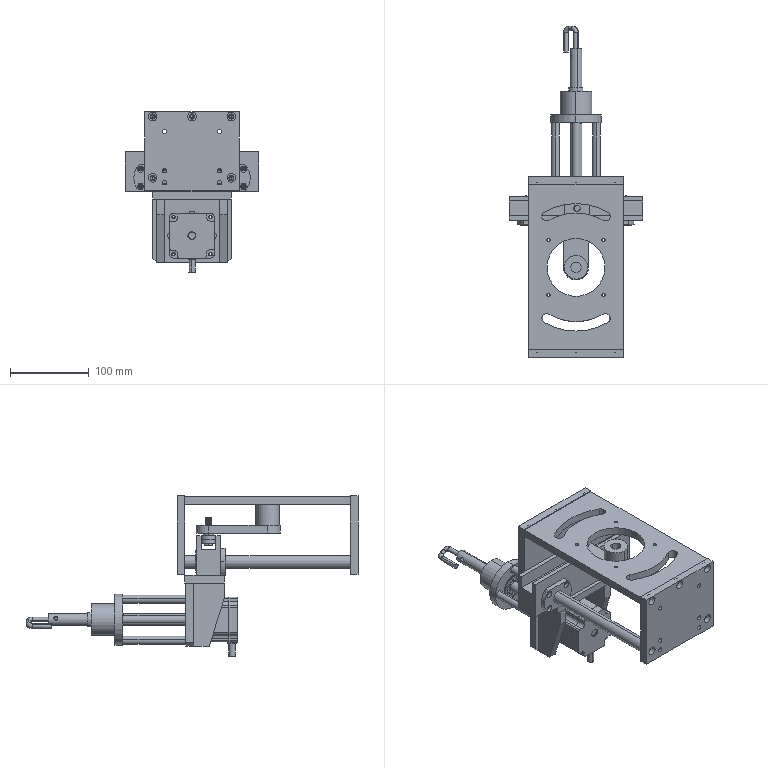Assembly | SolidWorks | mm | 28 component files | 28 solids | 1520 faces | box 170 x 421.99 x 203.93 mm | volume 1171784 mm3 | cylinder 610 | plane 329 | sphere 320 | torus 168 | cone 90 | spline 3 | commonest cylinder face diameters 10 x88 5.5 x60 4.2 x52 8 x50 5 x36 11 x32 6.6 x32 4.5 x24
Bill of materials:
75-02-11StirringUpperAndLowerMountingPlate | 2 | A3 Steel | Flat rectangular plate of uniform thickness with 11 round through holes: 5 larger holes (three across one long edge, two at the opposite corners) and 6 smaller holes in two columns placed inward of the larger ones.
75-02-12StirringMountingPlate | 1 | A3 Steel | Flat rectangular plate with a large central circular through hole, four small through holes around it, two curved (arc-shaped) slots with rounded ends on either side of the central hole, and three small holes drilled into one long edge face.
75-02-13StirringFixedOpticalAxis | 2 | A3 Steel | Long, slender, straight solid cylindrical rod with a small axial hole at the end.
75-02-14LinearBearingMountingPlate | 1 | A3 Steel | Rectangular block with a full-length rectangular channel cut along the top, giving a U-shaped cross-section. Two large round holes go through the side walls, each surrounded by four small holes in a square pattern.
75-02-15MotorSleeveAxis | 1 | A3 Steel | Thick-walled cylindrical sleeve (collar-like) with a central axial through bore and one small radial hole through the side wall.
75-02-16StirringConnectingRod | 1 | A3 Steel | Flat, obround (stadium-shaped) bar of uniform thickness with one round through hole near one rounded end and four smaller round through holes in a square/diamond pattern near the other end.
75-02-17StirringFixedEndAxis | 1 | A3 Steel | Stepped cylindrical stud/pin. From top to bottom: a threaded-looking section, a short reduced-diameter neck, a slightly larger shoulder, a larger plain cylindrical body, and a base flange with flats on two opposite sides.
75-02-18StirringMotorMountingPlateModified | 1 | A3 Steel | Flat rectangular plate of uniform thickness with 8 round through holes in a pattern symmetric about the plate's short axis, arranged in two mirrored groups of four.
75-02-19StirringMotorSupportPlate | 2 | A3 Steel | Prismatic bar of rectangular cross-section with one tapered side: its profile has a straight section near one end, then an angled face that narrows toward the other end. A single small hole is drilled into the wider end face.
75-02-20StirringMotorConnectionPlateModified | 1 | A3 Steel | Thick rectangular plate with two chamfered corners along one edge, a large central circular through hole, 12 surrounding through holes (4 large near the corners, 4 medium on the axes around the central hole, 4 small on the diagonals), and two holes drilled into the opposite edge face.
75-02-21StirringRod | 1 | A3 Steel | Long cylindrical shaft with a raised collar ring near one end, a faint circumferential line near the middle, a small cross (radial) hole near each end, and an axial hole at the end.
75-02-22MotorConnectingRod | 4 | A3 Steel | Straight cylindrical tube or rod of constant outside diameter with a concentric axial bore at the end.
75-02-23StirringBearingHousing | 1 | A3 Steel | Flanged cylindrical bushing-like part: thin circular flange with a longer cylindrical hub on one side, a central through bore, and four evenly spaced small through holes in the flange.
75-02-24RotatingHook | 1 | A3 Steel | Round rod of solid circular section bent 180 degrees into a hairpin/U shape with two parallel straight legs of unequal length and flat cut ends.
75-02-27ConnectingRodSpacer | 1 | A3 Steel | Plain flat annular ring (washer- or spacer-like) with a rectangular cross-section, concentric circular outer and inner edges, and flat parallel faces.
FlangeLinearBearingLMH16UU | 2 |  | Flanged cylindrical part with a truncated-circle flange (circular outline with two parallel flat sides), four through holes in the flange corners, a long cylindrical hub, and a central through bore.
GB_T276-94DeepGrooveBallBearing6002-2Z | 2 |  | Ring-type rolling-element assembly geometry: concentric outer and inner rings with a narrow annular gap in which spherical elements are partly visible. It resembles an open ball bearing.
GB_T276-94DeepGrooveBallBearing61800-2Z | 2 |  | Ring-type rolling-element assembly geometry similar to part-62d9...: outer ring and inner ring with spherical elements visible in the annular gap, plus a recessed groove ring on the face. It resembles a ball bearing.
X2_7535673A_X0_5756 | 1 | A3 Steel | Box-like motor-housing-shaped body with a square cross-section: a square front flange with rounded corners and four corner through holes, a raised circular pilot boss with a cylindrical shaft on the front face, and lengthwise relief grooves or chamfers along the body corners.
Mates:
1. coincident | 75-02-12StirringMountingPlate-1 face at (-77.8, 116.867, 112.75) dir (0, 1, 0) | 75-02-11StirringUpperAndLowerMountingPlate-1 face at (-17.8, 116.867, 63.75) dir (0, -1, 0)
2. concentric | 75-02-12StirringMountingPlate-1 face at (-67.8, 116.867, 107.75) dir (0, 1, 0) r 2.5 | 75-02-11StirringUpperAndLowerMountingPlate-1 face at (-67.8, 126.867, 107.75) dir (0, 1, 0) r 3.3
3. concentric | 75-02-12StirringMountingPlate-1 face at (-17.8, 116.867, 107.75) dir (0, 1, 0) r 2.5 | 75-02-11StirringUpperAndLowerMountingPlate-1 face at (-17.8, 126.867, 107.75) dir (0, 1, 0) r 3.3
4. coincident | 75-02-12StirringMountingPlate-1 face at (-77.8, -93.133, 112.75) dir (0, -1, 0) | 75-02-11StirringUpperAndLowerMountingPlate-2 face at (-17.8, -93.133, 63.75) dir (0, 1, 0)
5. concentric | 75-02-12StirringMountingPlate-1 face at (-67.8, -93.133, 107.75) dir (0, -1, 0) r 2.5 | 75-02-11StirringUpperAndLowerMountingPlate-2 face at (-67.8, -103.133, 107.75) dir (0, -1, 0) r 3.3
6. concentric | 75-02-12StirringMountingPlate-1 face at (32.2, -93.133, 107.75) dir (0, -1, 0) r 2.5 | 75-02-11StirringUpperAndLowerMountingPlate-2 face at (32.2, -103.133, 107.75) dir (0, -1, 0) r 3.3
7. concentric | 75-02-11StirringUpperAndLowerMountingPlate-1 face at (-67.8, 126.867, 29.75) dir (0, 1, 0) r 5.5 | 75-02-13StirringFixedOpticalAxis-1 face at (-67.8, 116.867, 29.75) dir (0, -1, 0) r 8
8. coincident | 75-02-11StirringUpperAndLowerMountingPlate-1 face at (-17.8, 116.867, 63.75) dir (0, -1, 0) | 75-02-13StirringFixedOpticalAxis-1 face at (-67.8, 116.867, 29.75) dir (0, 1, 0)
9. concentric | 75-02-11StirringUpperAndLowerMountingPlate-1 face at (32.2, 126.867, 29.75) dir (0, 1, 0) r 3.3 | 75-02-13StirringFixedOpticalAxis-2 face at (32.2, 116.867, 29.75) dir (0, -1, 0) r 8
10. coincident | 75-02-11StirringUpperAndLowerMountingPlate-1 face at (-17.8, 116.867, 63.75) dir (0, -1, 0) | 75-02-13StirringFixedOpticalAxis-2 face at (32.2, 116.867, 29.75) dir (0, 1, 0)
11. concentric | 75-02-13StirringFixedOpticalAxis-2 face at (32.2, 116.867, 29.75) dir (0, -1, 0) r 8 | FlangeLinearBearingLMH16UU-1 face at (32.2, 102.857, 29.75) dir (0, -1, 0) r 14
12. concentric | 75-02-13StirringFixedOpticalAxis-1 face at (-67.8, 116.867, 29.75) dir (0, -1, 0) r 8 | FlangeLinearBearingLMH16UU-2 face at (-67.8, 102.857, 29.75) dir (0, -1, 0) r 14
13. coincident | FlangeLinearBearingLMH16UU-1 face at (32.2, 71.857, 29.75) dir (0, 1, 0) | FlangeLinearBearingLMH16UU-2 face at (-67.8, 71.857, 29.75) dir (0, 1, 0)
14. concentric | 75-02-13StirringFixedOpticalAxis-2 face at (32.2, 116.867, 29.75) dir (0, -1, 0) r 8 | 75-02-14LinearBearingMountingPlate-1 face at (32.2, 101.857, 29.75) dir (0, -1, 0) r 14
15. concentric | 75-02-13StirringFixedOpticalAxis-1 face at (-67.8, 116.867, 29.75) dir (0, -1, 0) r 8 | 75-02-14LinearBearingMountingPlate-1 face at (-67.8, 101.857, 29.75) dir (0, -1, 0) r 14
16. coincident | FlangeLinearBearingLMH16UU-1 face at (32.2, 71.857, 29.75) dir (0, 1, 0) | 75-02-14LinearBearingMountingPlate-1 face at (67.2, 71.857, 62.75) dir (0, -1, 0)
17. concentric | FlangeLinearBearingLMH16UU-1 face at (16.7, 96.857, 18.75) dir (0, -1, 0) r 2.25 | 75-02-14LinearBearingMountingPlate-1 face at (16.7, 71.857, 18.75) dir (0, -1, 0) r 1.65
18. concentric | FlangeLinearBearingLMH16UU-2 face at (-52.3, 96.857, 18.75) dir (0, -1, 0) r 2.25 | 75-02-14LinearBearingMountingPlate-1 face at (-52.3, 71.857, 18.75) dir (0, -1, 0) r 1.65
19. coincident | 75-02-15MotorSleeveAxis-1 face at (-17.8, 11.867, 76.25) dir (0, 0, -1) | 75-02-16StirringConnectingRod-1 face at (-17.8, 11.867, 76.25) dir (0, 0, 1)
20. concentric | 75-02-15MotorSleeveAxis-1 face at (-7.802, 11.701, 76.25) dir (0, 0, -1) r 2.1 | 75-02-16StirringConnectingRod-1 face at (-7.802, 11.701, 66.25) dir (0, 0, -1) r 5
21. concentric | 75-02-15MotorSleeveAxis-1 face at (-17.634, 21.866, 76.25) dir (0, 0, -1) r 2.1 | 75-02-16StirringConnectingRod-1 face at (-17.634, 21.866, 66.25) dir (0, 0, -1) r 5
22. concentric | 75-02-16StirringConnectingRod-1 face at (-16.556, 86.857, 66.25) dir (0, 0, -1) r 3.4 | GB_T276-94DeepGrooveBallBearing61800-2Z-1 face at (-16.556, 86.857, 73.171) dir (0, 0, 1) r 5
23. concentric | GB_T276-94DeepGrooveBallBearing61800-2Z-1 face at (-16.556, 86.857, 60.75) dir (0, 0, 1) r 9.5 | GB_T276-94DeepGrooveBallBearing61800-2Z-2 face at (-16.556, 86.857, 55.75) dir (0, 0, 1) r 9.5
24. coincident | GB_T276-94DeepGrooveBallBearing61800-2Z-1 face at (-24.676, 82.533, 58.25) dir (0, 0, -1) | GB_T276-94DeepGrooveBallBearing61800-2Z-2 face at (-25.291, 83.971, 58.25) dir (0, 0, 1)
25. concentric | 75-02-16StirringConnectingRod-1 face at (-16.556, 86.857, 66.25) dir (0, 0, -1) r 3.4 | 75-02-27ConnectingRodSpacer-1 face at (-16.556, 86.857, 66.25) dir (0, 0, -1) r 6.5
26. coincident | 75-02-16StirringConnectingRod-1 face at (-17.8, 11.867, 66.25) dir (0, 0, -1) | 75-02-27ConnectingRodSpacer-1 face at (-16.556, 86.857, 66.25) dir (0, 0, 1)
27. coincident | GB_T276-94DeepGrooveBallBearing61800-2Z-1 face at (-22.117, 83.896, 63.25) dir (0, 0, 1) | 75-02-27ConnectingRodSpacer-1 face at (-16.556, 86.857, 63.25) dir (0, 0, -1)
28. tangent | 75-02-14LinearBearingMountingPlate-1 face at (67.2, 77.357, 45.75) dir (0, 1, 0) | GB_T276-94DeepGrooveBallBearing61800-2Z-1 face at (-16.556, 86.857, 60.75) dir (0, 0, 1) r 9.5
29. concentric | GB_T276-94DeepGrooveBallBearing61800-2Z-2 face at (-16.556, 86.857, 68.171) dir (0, 0, 1) r 5 | 75-02-17StirringFixedEndAxis-1 face at (-16.556, 86.857, 43.653) dir (0, 0, -1) r 5
30. coincident | GB_T276-94DeepGrooveBallBearing61800-2Z-2 face at (-22.538, 84.881, 53.25) dir (0, 0, -1) | 75-02-17StirringFixedEndAxis-1 face at (-16.556, 93.357, 53.25) dir (0, 0, 1)
31. concentric | 75-02-23StirringBearingHousing-1 face at (-17.87, 226.857, -43.68) dir (0, 1, 0) r 16 | GB_T276-94DeepGrooveBallBearing6002-2Z-1 face at (-17.87, 218.936, -43.68) dir (0, -1, 0) r 7.5
32. coincident | 75-02-23StirringBearingHousing-1 edge at (-17.87, 226.857, -43.68) dir (0, -1, 0) r 14 | GB_T276-94DeepGrooveBallBearing6002-2Z-1 face at (-20.936, 226.857, -59.078) dir (0, -1, 0)
33. concentric | 75-02-23StirringBearingHousing-1 face at (-17.87, 204.857, -43.68) dir (0, -1, 0) r 16 | GB_T276-94DeepGrooveBallBearing6002-2Z-2 face at (-17.87, 187.936, -43.68) dir (0, -1, 0) r 7.5
34. coincident | 75-02-23StirringBearingHousing-1 face at (-17.87, 204.857, -43.68) dir (0, -1, 0) | GB_T276-94DeepGrooveBallBearing6002-2Z-2 face at (-20.936, 204.857, -59.078) dir (0, 1, 0)
35. concentric | 75-02-21StirringRod-1 face at (-17.87, 78.734, -43.68) dir (0, -1, 0) r 7.5 | GB_T276-94DeepGrooveBallBearing6002-2Z-2 face at (-17.87, 187.936, -43.68) dir (0, -1, 0) r 7.5
36. coincident | 75-02-22MotorConnectingRod-1 face at (-17.8, 195.857, -17.75) dir (0, 1, 0) | 75-02-23StirringBearingHousing-1 face at (-17.87, 195.857, -43.68) dir (0, -1, 0)
37. coincident | 75-02-18StirringMotorMountingPlateModified-1 face at (-17.8, 91.857, 2.75) dir (0, 0, -1) | 75-02-20StirringMotorConnectionPlateModified-1 face at (-67.8, 115.857, 2.75) dir (0, 0, 1)
38. concentric | 75-02-18StirringMotorMountingPlateModified-1 face at (2.2, 110.857, 12.75) dir (0, 0, 1) r 5 | 75-02-20StirringMotorConnectionPlateModified-1 face at (2.2, 110.857, 2.75) dir (0, 0, 1) r 2.1
39. concentric | 75-02-18StirringMotorMountingPlateModified-1 face at (-37.8, 110.857, 12.75) dir (0, 0, 1) r 5 | 75-02-20StirringMotorConnectionPlateModified-1 face at (-37.8, 110.857, 2.75) dir (0, 0, 1) r 2.1
40. coincident | X2_7535673A_X0_5756-1 face at (-17.87, 105.857, -43.68) dir (0, 1, 0) | 75-02-20StirringMotorConnectionPlateModified-1 face at (-17.8, 105.857, -37.25) dir (0, -1, 0)
41. concentric | X2_7535673A_X0_5756-1 face at (5.7, 102.857, -67.25) dir (0, 1, 0) r 2.25 | 75-02-20StirringMotorConnectionPlateModified-1 face at (5.7, 115.857, -67.25) dir (0, 1, 0) r 1.65
42. parallel | X2_7535673A_X0_5756-1 face at (-46.37, 100.357, -43.68) dir (-1, 0, 0) | 75-02-20StirringMotorConnectionPlateModified-1 face at (-67.8, 115.857, 2.75) dir (-1, 0, 0)
43. coincident | 75-02-20StirringMotorConnectionPlateModified-1 face at (-17.8, 115.857, -37.25) dir (0, 1, 0) | 75-02-22MotorConnectingRod-1 face at (-17.8, 115.857, -17.75) dir (0, -1, 0)
44. concentric | X2_7535673A_X0_5756-1 face at (-17.87, 115.357, -43.68) dir (0, -1, 0) r 3.175 | 75-02-21StirringRod-1 face at (-17.87, 78.734, -43.68) dir (0, -1, 0) r 7.5
45. concentric | 75-02-20StirringMotorConnectionPlateModified-1 face at (-17.8, 105.857, -17.75) dir (0, -1, 0) r 2.75 | 75-02-22MotorConnectingRod-1 face at (-17.8, 115.857, -17.75) dir (0, 1, 0) r 5
46. parallel | 75-02-18StirringMotorMountingPlateModified-1 face at (-67.8, 116.857, 2.75) dir (-1, 0, 0) | 75-02-23StirringBearingHousing-1 plane at (-17.87, 205.857, -43.68) dir (-1, 0, 0)
47. coincident | 75-02-21StirringRod-1 face at (-10.635, 235.857, -45.654) dir (0, -1, 0) | GB_T276-94DeepGrooveBallBearing6002-2Z-1 face at (-19.862, 235.857, -53.684) dir (0, 1, 0)
48. coincident | 75-02-18StirringMotorMountingPlateModified-1 face at (-17.8, 91.857, 2.75) dir (0, 0, -1) | 75-02-19StirringMotorSupportPlate-1 face at (17.2, 66.857, 2.75) dir (0, 0, 1)
49. coincident | 75-02-20StirringMotorConnectionPlateModified-1 face at (-17.8, 105.857, -37.25) dir (0, -1, 0) | 75-02-19StirringMotorSupportPlate-1 face at (17.2, 105.857, 2.75) dir (0, 1, 0)
50. concentric | 75-02-18StirringMotorMountingPlateModified-1 face at (22.2, 86.857, 12.75) dir (0, 0, 1) r 5.5 | 75-02-19StirringMotorSupportPlate-1 face at (22.2, 86.857, 2.75) dir (0, 0, 1) r 2.5
51. coincident | 75-02-18StirringMotorMountingPlateModified-1 face at (-17.8, 91.857, 2.75) dir (0, 0, -1) | 75-02-19StirringMotorSupportPlate-2 face at (-62.8, 66.857, 2.75) dir (0, 0, 1)
52. coincident | 75-02-20StirringMotorConnectionPlateModified-1 face at (-17.8, 105.857, -37.25) dir (0, -1, 0) | 75-02-19StirringMotorSupportPlate-2 face at (-62.8, 105.857, 2.75) dir (0, 1, 0)
53. concentric | 75-02-20StirringMotorConnectionPlateModified-1 face at (-57.8, 115.857, -17.25) dir (0, 1, 0) r 3.3 | 75-02-19StirringMotorSupportPlate-2 face at (-57.8, 105.857, -17.25) dir (0, 1, 0) r 2.5
54. coincident | 75-02-14LinearBearingMountingPlate-1 face at (-17.8, 86.857, 12.75) dir (0, 0, -1) | 75-02-18StirringMotorMountingPlateModified-1 face at (-17.8, 91.857, 12.75) dir (0, 0, 1)
55. concentric | 75-02-14LinearBearingMountingPlate-1 face at (-45.3, 76.857, 12.75) dir (0, 0, -1) r 2.1 | 75-02-18StirringMotorMountingPlateModified-1 face at (-45.3, 76.857, 2.75) dir (0, 0, -1) r 5
56. concentric | 75-02-14LinearBearingMountingPlate-1 face at (9.7, 96.857, 12.75) dir (0, 0, -1) r 2.1 | 75-02-18StirringMotorMountingPlateModified-1 face at (9.7, 96.857, 2.75) dir (0, 0, -1) r 5
57. concentric | 75-02-21StirringRod-1 face at (-17.87, 260.857, -43.68) dir (0, 1, 0) r 3 | 75-02-24RotatingHook-1 face at (-17.87, 265.857, -43.68) dir (0, 1, 0) r 3
58. distance | 75-02-24RotatingHook-1 face at (-17.87, 265.857, -43.68) dir (0, -1, 0) | 75-02-21StirringRod-1 face at (-10.635, 290.857, -45.654) dir (0, 1, 0)